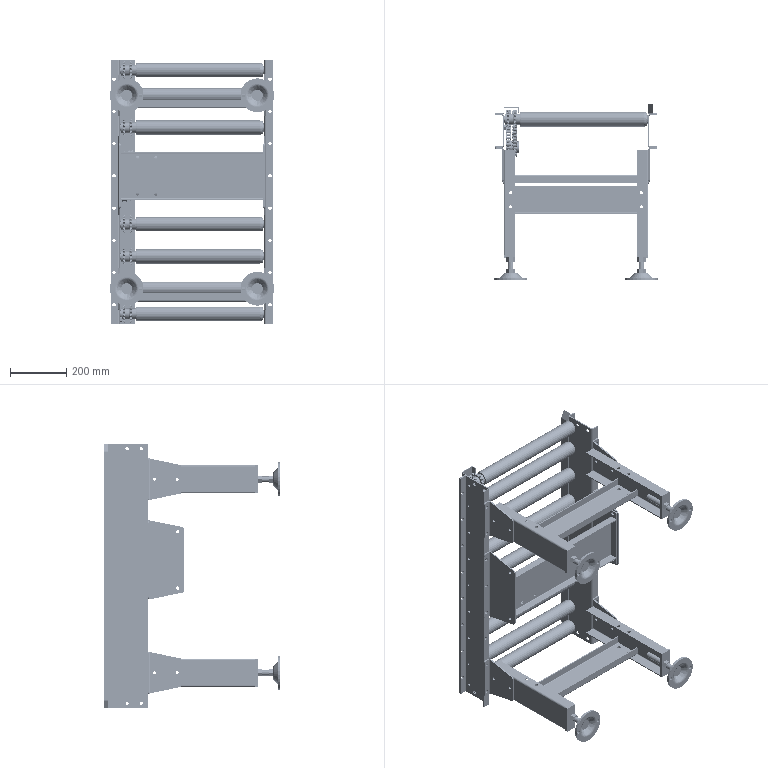Assembly | SolidWorks | mm | 34 component files | 142 solids | 9051 faces | box 583 x 625 x 935 mm | volume 14049367 mm3 | cylinder 4520 | plane 2988 | spline 894 | cone 551 | torus 98 | commonest cylinder face diameters 32.678 x540 4.45 x512 8.596 x396 11.81 x384 12 x276 63.6 x270 57.066 x256 30.1 x153
Bill of materials:
Default | 1 |  | Closed-loop single-strand roller chain in an elongated oval/racetrack path.
08B-2Chain32Links | 1 |  | Closed-loop roller-chain-style link band laid out in an elongated oval/stadium path, made of repeating alternating side plates joined by pins with cylindrical rollers between the plates.
BF-20AdjustableCupFoot | 4 | Q235A | Leveling-foot-like part: a circular flanged base with a conical raised center, plus a straight cylindrical rod with two hex sections.
GB_T41-20001HexNutCGradeM10 | 1 | Grade 4 | Hexagonal nut with a plain central bore and chamfered corners on both faces.
JGS01-0001EndCorner | 4 | Plain Carbon Steel | Bent sheet-metal L-bracket with a trapezoidal main flange and a narrow short flange, two holes in each.
JGS01-0002ConveyorLeg1 | 4 | Plain Carbon Steel | Elongated channel-type profile with a thickened block or plate at one end containing a large round hole, and small holes in the flanges and web.
05B | 1 |  | Double sprocket-like toothed wheel: two identical spaced toothed rims on one cylindrical hub, with the hub extending past one rim, a plain round through-bore, and small radial holes in the extended hub.
JGS01-0004DriveFixingBracket | 2 | Plain Carbon Steel | Bent sheet-metal L-bracket with a tapered main flange holding two holes and a narrow return flange holding three holes.
JGS02-0001LegTieRod2 | 2 | Plain Carbon Steel | Long, shallow U-channel sheet-metal part with rounded bends and four holes in the base, two near each end.
JGS02-0002ConveyorMotorMountingPlate2 | 1 | Plain Carbon Steel | Channel-section beam with flat end tabs at both ends, each tab carrying two holes, and four holes in the web near one end.
JGS02-0003Guardrail2 | 1 | Plain Carbon Steel | Long, slender angle-section (L-profile) strip with one row of holes along one leg and angled, chamfered ends.
2.224.JHA.ACC-450W | 9 |  | Cylindrical tube roller with a double sprocket (two toothed rings) at one end and a domed end cap at the other.
JGS02-A0001RollerBracket2 | 2 | Plain Carbon Steel | Long C-channel (lipless U-section) with holes in the web and both flanges along its length.
JGS02-A0002ChainGuard2 | 1 | Plain Carbon Steel | Long formed sheet-metal profile with a stepped hat/Z-like cross-section: an offset flat flange, a raised web, and a downturned leg, with holes along one face.
Mates:
1. coincident | JGS02-A0000RollerAssembly2-1/JGS02-A0001RollerBracket2-2 face at (-169.116, 34.367, -467.5) dir (0, -1, 0) | JGS01-0001EndCorner-1 face at (-169.116, 34.367, 342.9) dir (0, 1, 0)
2. coincident | JGS02-A0000RollerAssembly2-1/JGS02-A0001RollerBracket2-2 face at (-199.116, 38.367, -467.5) dir (-1, 0, 0) | JGS01-0001EndCorner-1 face at (-199.116, 34.367, 417.9) dir (-1, 0, 0)
3. concentric | JGS02-A0000RollerAssembly2-1/JGS02-A0001RollerBracket2-2 face at (-189.116, 154.367, 400.05) dir (0, 1, 0) r 6 | JGS01-0001EndCorner-1 face at (-189.116, 29.367, 400.05) dir (0, 1, 0) r 6
4. coincident | JGS02-A0000RollerAssembly2-1/JGS02-A0001RollerBracket2-1 face at (343.884, 34.367, 467.5) dir (0, -1, 0) | JGS01-0001EndCorner-5 face at (343.884, 34.367, 342.9) dir (0, 1, 0)
5. coincident | JGS02-A0000RollerAssembly2-1/JGS02-A0001RollerBracket2-1 face at (373.884, 38.367, 467.5) dir (1, 0, 0) | JGS01-0001EndCorner-5 face at (373.884, 34.367, 267.9) dir (1, 0, 0)
6. concentric | 08B-2Chain32Links-1 sketch segment at (-130.112, 134.367, 114.3) dir (-1, 0, 0) r 28.537 | JGS02-A0000RollerAssembly2-1/2.224.JHA.ACC-450W-32 face at (342.884, 134.367, 114.3) dir (1, 0, 0) r 25.3
7. concentric | JGS02-A0000RollerAssembly2-1/2.224.JHA.ACC-450W-31 face at (342.884, 134.367, 0) dir (1, 0, 0) r 25.3 | 08B-2Chain32Links-2 sketch segment at (-152.112, 134.367, 0) dir (-1, 0, 0) r 28.537
8. coincident | JGS02-A0000RollerAssembly2-1/JGS02-A0001RollerBracket2-2 face at (-169.116, 34.367, -467.5) dir (0, -1, 0) | JGS01-0004DriveFixingBracket-1 face at (-169.116, 34.367, 57.15) dir (0, 1, 0)
9. coincident | JGS02-A0000RollerAssembly2-1/JGS02-A0001RollerBracket2-2 face at (-199.116, 38.367, -467.5) dir (-1, 0, 0) | JGS01-0004DriveFixingBracket-1 face at (-199.116, 34.367, 197.15) dir (-1, 0, 0)
10. coincident | JGS02-0002ConveyorMotorMountingPlate2-1 face at (-169.116, -87.12, 164.65) dir (-1, 0, 0) | JGS01-0004DriveFixingBracket-1 face at (-169.116, -30.633, 57.15) dir (1, 0, 0)
11. coincident | JGS02-A0000RollerAssembly2-1/JGS02-A0001RollerBracket2-1 face at (343.884, 34.367, 467.5) dir (0, -1, 0) | JGS01-0004DriveFixingBracket-2 face at (343.884, 34.367, 57.15) dir (0, 1, 0)
12. concentric | JGS02-A0000RollerAssembly2-1/JGS02-A0001RollerBracket2-2 face at (-173.116, 106.867, -451.5) dir (-1, 0, 0) r 6 | GB_T41-20001HexNutCGradeM10-1 face at (-169.116, 106.867, -451.5) dir (1, 0, 0) r 5
13. coincident | JGS02-A0000RollerAssembly2-1/JGS02-A0001RollerBracket2-2 face at (-169.116, 154.367, -467.5) dir (1, 0, 0) | GB_T41-20001HexNutCGradeM10-1 face at (-169.116, 114.483, -447.103) dir (-1, 0, 0)
14. coincident | JGS02-A0000RollerAssembly2-1/JGS02-A0001RollerBracket2-2 face at (-173.116, 154.367, -467.5) dir (-1, 0, 0) | assembly face at (-173.116, 44.367, -467.5) dir (1, 0, 0)
15. concentric | JGS02-A0000RollerAssembly2-1/JGS02-A0001RollerBracket2-2 face at (-173.116, 56.867, -451.5) dir (-1, 0, 0) r 6 | assembly face at (-173.116, 56.867, -453.5) dir (-1, 0, 0) r 5
16. coincident | JGS02-A0000RollerAssembly2-1/JGS02-A0001RollerBracket2-1 face at (347.884, 154.367, 467.5) dir (1, 0, 0) | assembly face at (347.884, 144.367, -467.5) dir (-1, 0, 0)
17. concentric | JGS02-A0000RollerAssembly2-1/JGS02-A0001RollerBracket2-1 face at (347.884, 106.867, -451.5) dir (1, 0, 0) r 6 | assembly face at (347.884, 106.867, -453.5) dir (1, 0, 0) r 5
18. concentric | JGS02-A0000RollerAssembly2-1/JGS02-A0001RollerBracket2-1 face at (347.884, 56.867, -451.5) dir (1, 0, 0) r 6 | assembly face at (347.884, 56.867, -453.5) dir (1, 0, 0) r 5
19. coincident | JGS02-A0000RollerAssembly2-1/JGS02-A0001RollerBracket2-1 face at (373.884, 154.367, 467.5) dir (0, 1, 0) | JGS02-0003Guardrail2-1 face at (343.884, 154.367, 0) dir (0, -1, 0)
20. concentric | JGS02-A0000RollerAssembly2-1/JGS02-A0001RollerBracket2-1 face at (363.884, 154.367, -400.05) dir (0, 1, 0) r 6 | JGS02-0003Guardrail2-1 face at (363.884, 154.367, -400.05) dir (0, 1, 0) r 6
21. coincident | JGS02-A0000RollerAssembly2-1/JGS02-A0001RollerBracket2-1 face at (373.884, 154.367, 467.5) dir (1, 0, 0) | JGS02-0003Guardrail2-1 face at (373.884, 154.367, 440.715) dir (1, 0, 0)
22. coincident | JGS01-0001EndCorner-1 face at (-169.116, -85.633, 342.9) dir (1, 0, 0) | JGS01-0002ConveyorLeg1-1 face at (-169.116, 24.367, 292.9) dir (-1, 0, 0)
23. coincident | JGS01-0001EndCorner-1 edge at (-169.116, 9.367, 342.9) dir (1, 0, 0) r 5.25 | JGS01-0002ConveyorLeg1-1 face at (-165.116, 9.367, 342.9) dir (-1, 0, 0) r 5.25
24. concentric | JGS01-0001EndCorner-1 face at (-174.116, -70.633, 342.9) dir (1, 0, 0) r 5.25 | JGS01-0002ConveyorLeg1-1 face at (-165.116, -70.633, 342.9) dir (-1, 0, 0) r 5.25
25. concentric | BF-20AdjustableCupFoot-1 face at (-144.116, -410.633, 342.9) dir (0, -1, 0) r 10 | JGS01-0002ConveyorLeg1-1 face at (-144.116, -355.633, 342.9) dir (0, -1, 0) r 10
26. coincident | BF-20AdjustableCupFoot-1 face at (-144.116, -355.633, 342.9) dir (0, 1, 0) | JGS01-0002ConveyorLeg1-1 face at (-169.116, -355.633, 342.9) dir (0, -1, 0)
27. coincident | JGS01-0001EndCorner-5 face at (343.884, -85.633, 342.9) dir (-1, 0, 0) | JGS01-0002ConveyorLeg1-4 face at (343.884, 24.367, 392.9) dir (1, 0, 0)
28. concentric | JGS01-0001EndCorner-5 face at (348.884, 9.367, 342.9) dir (-1, 0, 0) r 5.25 | JGS01-0002ConveyorLeg1-4 face at (339.884, 9.367, 342.9) dir (1, 0, 0) r 5.25
29. concentric | JGS01-0001EndCorner-5 face at (348.884, -70.633, 342.9) dir (-1, 0, 0) r 5.25 | JGS01-0002ConveyorLeg1-4 face at (339.884, -70.633, 342.9) dir (1, 0, 0) r 5.25
30. concentric | BF-20AdjustableCupFoot-4 face at (318.884, -410.633, 342.9) dir (0, -1, 0) r 10 | JGS01-0002ConveyorLeg1-4 face at (318.884, -355.633, 342.9) dir (0, -1, 0) r 10
31. coincident | BF-20AdjustableCupFoot-4 face at (318.884, -355.633, 342.9) dir (0, 1, 0) | JGS01-0002ConveyorLeg1-4 face at (343.884, -355.633, 342.9) dir (0, -1, 0)
32. coincident | JGS01-0002ConveyorLeg1-1 face at (-129.116, 24.367, 296.9) dir (0, 0, 1) | JGS02-0001LegTieRod2-1 face at (-162.616, -100.633, 296.9) dir (0, 0, -1)
33. concentric | JGS01-0002ConveyorLeg1-1 face at (-144.116, -125.633, 292.9) dir (0, 0, 1) r 6 | JGS02-0001LegTieRod2-1 face at (-144.116, -125.633, 300.9) dir (0, 0, -1) r 6
34. concentric | JGS01-0002ConveyorLeg1-1 face at (-144.116, -175.633, 292.9) dir (0, 0, 1) r 6 | JGS02-0001LegTieRod2-1 face at (-144.116, -175.633, 300.9) dir (0, 0, -1) r 6
35. coincident | JGS02-0002ConveyorMotorMountingPlate2-1 face at (343.884, -87.12, 164.65) dir (1, 0, 0) | JGS01-0004DriveFixingBracket-2 face at (343.884, -30.633, 57.15) dir (-1, 0, 0)
36. concentric | JGS02-A0000RollerAssembly2-1/JGS02-A0001RollerBracket2-1 face at (363.884, 154.367, 57.15) dir (0, 1, 0) r 6 | JGS01-0004DriveFixingBracket-2 face at (363.884, 30.367, 57.15) dir (0, 1, 0) r 6
37. parallel | JGS02-A0000RollerAssembly2-1/JGS02-A0001RollerBracket2-2 face at (-169.116, 34.367, -467.5) dir (0, -1, 0) | JGS02-0002ConveyorMotorMountingPlate2-1 face at (87.384, -62.12, 57.15) dir (0, 1, 0)
38. concentric | JGS02-A0000RollerAssembly2-1/JGS02-A0001RollerBracket2-1 face at (363.884, 154.367, 400.05) dir (0, 1, 0) r 6 | JGS01-0001EndCorner-5 face at (363.884, 29.367, 400.05) dir (0, 1, 0) r 6
39. distance | 08B-2Chain32Links-1 face at (-126.237, 139.451, 104.152) dir (-1, 0, 0) | JGS02-A0000RollerAssembly2-1/2.224.JHA.ACC-450W-32 face at (-126.591, 134.367, 114.3) dir (1, 0, 0)
40. distance | 08B-2Chain32Links-1 face at (-126.237, 48.821, 78.32) dir (-1, 0, 0) | JGS01-000308B14TSprocket-1 face at (-126.508, 58.583, 64.307) dir (1, 0, 0)
41. distance | 08B-2Chain32Links-2 face at (-148.237, 69.161, 24.605) dir (-1, 0, 0) | JGS02-A0000RollerAssembly2-1/2.224.JHA.ACC-450W-32 face at (-148.591, 134.367, 114.3) dir (1, 0, 0)
42. coincident | JGS02-A0001RollerBracket2-2 face at (-548.341, 63.834, -467.5) dir (1, 0, 0) | 2.224.JHA.ACC-450W-1 face at (-548.341, 43.834, -431.8) dir (-1, 0, 0)
43. concentric | 2.224.JHA.ACC-450W-1 face at (-36.341, 43.834, -431.8) dir (1, 0, 0) r 25.3 | JGS02-A0001RollerBracket2-2 face at (-548.341, 43.834, -431.8) dir (-1, 0, 0) r 4.25
44. coincident | 2.224.JHA.ACC-450W-1 face at (-35.341, 43.834, -431.8) dir (1, 0, 0) | JGS02-A0001RollerBracket2-1 face at (-35.341, 63.834, 467.5) dir (-1, 0, 0)
45. concentric | 2.224.JHA.ACC-450W-1 face at (-35.341, 43.834, -431.8) dir (1, 0, 0) r 3.4 | JGS02-A0001RollerBracket2-2 face at (-548.341, 43.834, -431.8) dir (-1, 0, 0) r 4.25
46. coincident | JGS02-A0001RollerBracket2-1 face at (-5.341, 63.834, 467.5) dir (0, 1, 0) | JGS02-A0001RollerBracket2-2 face at (-578.341, 63.834, -467.5) dir (0, 1, 0)
47. coincident | JGS02-A0001RollerBracket2-2 face at (-578.341, 63.834, -467.5) dir (0, 1, 0) | JGS02-A0002ChainGuard2-1 face at (-578.341, 63.834, 467.5) dir (0, -1, 0)
48. coincident | JGS02-A0001RollerBracket2-2 face at (-554.341, -50.166, 467.5) dir (0, 0, 1) | JGS02-A0002ChainGuard2-1 face at (-548.341, 66.834, 467.5) dir (0, 0, 1)
49. coincident | JGS02-A0001RollerBracket2-2 face at (-578.341, 63.834, -467.5) dir (-1, 0, 0) | JGS02-A0002ChainGuard2-1 face at (-578.341, 63.834, 467.5) dir (-1, 0, 0)
50. concentric | JGS02-A0001RollerBracket2-1 face at (-35.341, 43.834, -342.9) dir (1, 0, 0) r 4.25 | 2.224.JHA.ACC-450W-28 face at (-36.341, 43.834, -342.9) dir (1, 0, 0) r 25.3
51. coincident | JGS02-A0001RollerBracket2-1 face at (-35.341, 63.834, 467.5) dir (-1, 0, 0) | 2.224.JHA.ACC-450W-28 face at (-35.341, 43.834, -342.9) dir (1, 0, 0)
52. concentric | JGS02-A0001RollerBracket2-1 face at (-35.341, 43.834, 431.8) dir (1, 0, 0) r 4.25 | 2.224.JHA.ACC-450W-35 face at (-36.341, 43.834, 431.8) dir (1, 0, 0) r 25.3
53. coincident | JGS02-A0001RollerBracket2-1 face at (-35.341, 63.834, 467.5) dir (-1, 0, 0) | 2.224.JHA.ACC-450W-35 face at (-35.341, 43.834, 431.8) dir (1, 0, 0)